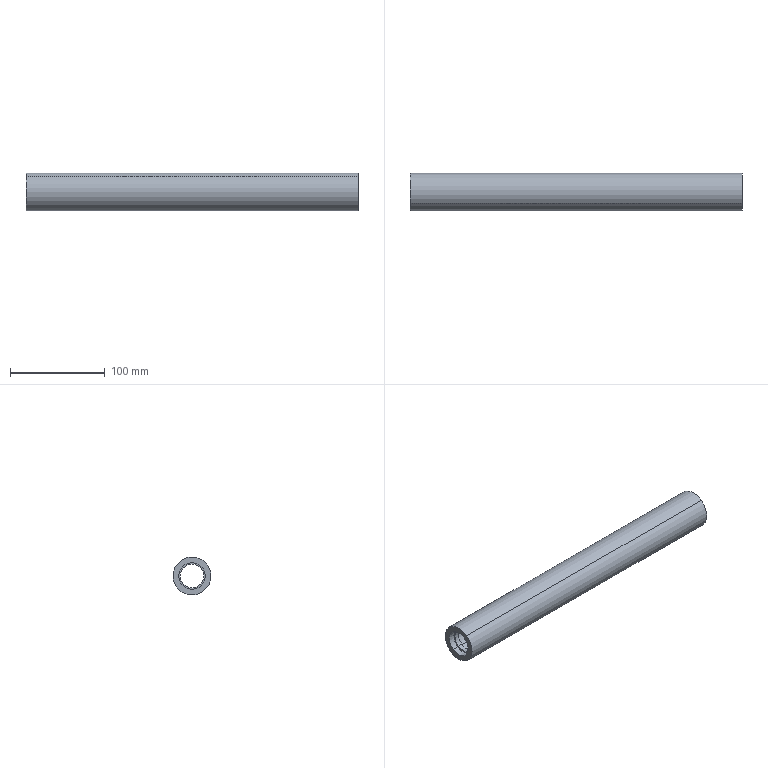Component | SolidWorks | 01-10MarkingMachineIdlerRoller-2 | 1 solid | 18 faces | box 350 x 40 x 40 mm | volume 130312 mm3 | cylinder 12 | plane 6 | commonest cylinder face diameters 28 x4 25 x4 40 x2 34 x2 | material A3 Steel
build123d program:
from build123d import *


with BuildPart() as part:
    # Sketch1 → Revolve1 (revolve)
    with BuildSketch(Plane.XY, mode=Mode.PRIVATE) as revolve1_sk:
        Polygon((-175, 20), (175, 20), (175, 14), (168, 14), (168, 12.5), (163, 12.5), (163, 17), (-163, 17), (-163, 12.5), (-168, 12.5), (-168, 14), (-175, 14), align=None)
    revolve(revolve1_sk.sketch.rotate(Axis((-220.554, 0, 0), (1, 0, 0)), 90), axis=Axis((-220.554, 0, 0), (1, 0, 0)))


solid = part.part

# Placed as in the assembly
solid = solid.moved(Location((-256.91, 57.41, 27.5), (0, 0, 0)))
STEP:
#1=COLOUR_RGB('',0.7922,0.8196,0.9333);
#2=FILL_AREA_STYLE_COLOUR('',#1);
#3=FILL_AREA_STYLE('',(#2));
#4=SURFACE_STYLE_FILL_AREA(#3);
#5=SURFACE_SIDE_STYLE('',(#4));
#6=SURFACE_STYLE_USAGE(.BOTH.,#5);
#7=PRESENTATION_STYLE_ASSIGNMENT((#6));
#8=CARTESIAN_POINT('',(-3.225,1.798,1.72));
#9=VERTEX_POINT('',#8);
#10=CARTESIAN_POINT('',(-3.225,2.722,0.4451));
#11=VERTEX_POINT('',#10);
#12=CARTESIAN_POINT('',(-3.225,2.26,1.083));
#13=DIRECTION('',(-1.,0.,0.));
#14=DIRECTION('',(0.,-0.5868,0.8097));
#15=AXIS2_PLACEMENT_3D('',#12,#13,#14);
#16=CIRCLE('',#15,0.7874);
#17=EDGE_CURVE('',#9,#11,#16,.T.);
#18=ORIENTED_EDGE('',*,*,#17,.T.);
#19=CARTESIAN_POINT('',(-17.004,2.722,0.4451));
#20=VERTEX_POINT('',#19);
#21=CARTESIAN_POINT('',(-18.798,2.722,0.4451));
#22=DIRECTION('',(-1.,0.,0.));
#23=VECTOR('',#22,39.37);
#24=LINE('',#21,#23);
#25=EDGE_CURVE('',#11,#20,#24,.T.);
#26=ORIENTED_EDGE('',*,*,#25,.T.);
#27=CARTESIAN_POINT('',(-17.004,1.798,1.72));
#28=VERTEX_POINT('',#27);
#29=CARTESIAN_POINT('',(-17.004,2.26,1.083));
#30=DIRECTION('',(-1.,0.,0.));
#31=DIRECTION('',(0.,-0.5868,0.8097));
#32=AXIS2_PLACEMENT_3D('',#29,#30,#31);
#33=CIRCLE('',#32,0.7874);
#34=EDGE_CURVE('',#28,#20,#33,.T.);
#35=ORIENTED_EDGE('',*,*,#34,.F.);
#36=CARTESIAN_POINT('',(-18.798,1.798,1.72));
#37=DIRECTION('',(-1.,0.,0.));
#38=VECTOR('',#37,39.37);
#39=LINE('',#36,#38);
#40=EDGE_CURVE('',#9,#28,#39,.T.);
#41=ORIENTED_EDGE('',*,*,#40,.F.);
#42=EDGE_LOOP('',(#18,#26,#35,#41));
#43=FACE_OUTER_BOUND('',#42,.T.);
#44=CARTESIAN_POINT('',(-18.798,2.26,1.083));
#45=DIRECTION('',(-1.,0.,0.));
#46=DIRECTION('',(0.,-0.5868,0.8097));
#47=AXIS2_PLACEMENT_3D('',#44,#45,#46);
#48=CYLINDRICAL_SURFACE('',#47,0.7874);
#49=ADVANCED_FACE('',(#43),#48,.T.);
#50=CARTESIAN_POINT('',(-3.225,2.584,0.6364));
#51=VERTEX_POINT('',#50);
#52=CARTESIAN_POINT('',(-3.225,1.937,1.529));
#53=VERTEX_POINT('',#52);
#54=CARTESIAN_POINT('',(-3.225,2.26,1.083));
#55=DIRECTION('',(-1.,0.,0.));
#56=DIRECTION('',(0.,-0.5868,0.8097));
#57=AXIS2_PLACEMENT_3D('',#54,#55,#56);
#58=CIRCLE('',#57,0.5512);
#59=EDGE_CURVE('',#51,#53,#58,.T.);
#60=ORIENTED_EDGE('',*,*,#59,.F.);
#61=CARTESIAN_POINT('',(-3.5,2.584,0.6364));
#62=VERTEX_POINT('',#61);
#63=CARTESIAN_POINT('',(-18.798,2.584,0.6364));
#64=DIRECTION('',(-1.,0.,0.));
#65=VECTOR('',#64,39.37);
#66=LINE('',#63,#65);
#67=EDGE_CURVE('',#51,#62,#66,.T.);
#68=ORIENTED_EDGE('',*,*,#67,.T.);
#69=CARTESIAN_POINT('',(-3.5,1.937,1.529));
#70=VERTEX_POINT('',#69);
#71=CARTESIAN_POINT('',(-3.5,2.26,1.083));
#72=DIRECTION('',(-1.,0.,0.));
#73=DIRECTION('',(0.,-0.5868,0.8097));
#74=AXIS2_PLACEMENT_3D('',#71,#72,#73);
#75=CIRCLE('',#74,0.5512);
#76=EDGE_CURVE('',#62,#70,#75,.T.);
#77=ORIENTED_EDGE('',*,*,#76,.T.);
#78=CARTESIAN_POINT('',(-18.798,1.937,1.529));
#79=DIRECTION('',(-1.,0.,0.));
#80=VECTOR('',#79,39.37);
#81=LINE('',#78,#80);
#82=EDGE_CURVE('',#53,#70,#81,.T.);
#83=ORIENTED_EDGE('',*,*,#82,.F.);
#84=EDGE_LOOP('',(#60,#68,#77,#83));
#85=FACE_OUTER_BOUND('',#84,.T.);
#86=CARTESIAN_POINT('',(-18.798,2.26,1.083));
#87=DIRECTION('',(-1.,0.,0.));
#88=DIRECTION('',(0.,-0.5868,0.8097));
#89=AXIS2_PLACEMENT_3D('',#86,#87,#88);
#90=CYLINDRICAL_SURFACE('',#89,0.5512);
#91=ADVANCED_FACE('',(#85),#90,.F.);
#92=CARTESIAN_POINT('',(-3.5,2.549,0.6842));
#93=VERTEX_POINT('',#92);
#94=CARTESIAN_POINT('',(-3.5,1.971,1.481));
#95=VERTEX_POINT('',#94);
#96=CARTESIAN_POINT('',(-3.5,2.26,1.083));
#97=DIRECTION('',(-1.,0.,0.));
#98=DIRECTION('',(0.,-0.5868,0.8097));
#99=AXIS2_PLACEMENT_3D('',#96,#97,#98);
#100=CIRCLE('',#99,0.4921);
#101=EDGE_CURVE('',#93,#95,#100,.T.);
#102=ORIENTED_EDGE('',*,*,#101,.F.);
#103=CARTESIAN_POINT('',(-3.697,2.549,0.6842));
#104=VERTEX_POINT('',#103);
#105=CARTESIAN_POINT('',(-18.798,2.549,0.6842));
#106=DIRECTION('',(-1.,0.,0.));
#107=VECTOR('',#106,39.37);
#108=LINE('',#105,#107);
#109=EDGE_CURVE('',#93,#104,#108,.T.);
#110=ORIENTED_EDGE('',*,*,#109,.T.);
#111=CARTESIAN_POINT('',(-3.697,1.971,1.481));
#112=VERTEX_POINT('',#111);
#113=CARTESIAN_POINT('',(-3.697,2.26,1.083));
#114=DIRECTION('',(-1.,0.,0.));
#115=DIRECTION('',(0.,-0.5868,0.8097));
#116=AXIS2_PLACEMENT_3D('',#113,#114,#115);
#117=CIRCLE('',#116,0.4921);
#118=EDGE_CURVE('',#104,#112,#117,.T.);
#119=ORIENTED_EDGE('',*,*,#118,.T.);
#120=CARTESIAN_POINT('',(-18.798,1.971,1.481));
#121=DIRECTION('',(-1.,0.,0.));
#122=VECTOR('',#121,39.37);
#123=LINE('',#120,#122);
#124=EDGE_CURVE('',#95,#112,#123,.T.);
#125=ORIENTED_EDGE('',*,*,#124,.F.);
#126=EDGE_LOOP('',(#102,#110,#119,#125));
#127=FACE_OUTER_BOUND('',#126,.T.);
#128=CARTESIAN_POINT('',(-18.798,2.26,1.083));
#129=DIRECTION('',(-1.,0.,0.));
#130=DIRECTION('',(0.,-0.5868,0.8097));
#131=AXIS2_PLACEMENT_3D('',#128,#129,#130);
#132=CYLINDRICAL_SURFACE('',#131,0.4921);
#133=ADVANCED_FACE('',(#127),#132,.F.);
#134=CARTESIAN_POINT('',(-3.697,2.653,0.5407));
#135=VERTEX_POINT('',#134);
#136=CARTESIAN_POINT('',(-3.697,1.867,1.625));
#137=VERTEX_POINT('',#136);
#138=CARTESIAN_POINT('',(-3.697,2.26,1.083));
#139=DIRECTION('',(-1.,0.,0.));
#140=DIRECTION('',(0.,-0.5868,0.8097));
#141=AXIS2_PLACEMENT_3D('',#138,#139,#140);
#142=CIRCLE('',#141,0.6693);
#143=EDGE_CURVE('',#135,#137,#142,.T.);
#144=ORIENTED_EDGE('',*,*,#143,.F.);
#145=CARTESIAN_POINT('',(-16.532,2.653,0.5407));
#146=VERTEX_POINT('',#145);
#147=CARTESIAN_POINT('',(-18.798,2.653,0.5407));
#148=DIRECTION('',(-1.,0.,0.));
#149=VECTOR('',#148,39.37);
#150=LINE('',#147,#149);
#151=EDGE_CURVE('',#135,#146,#150,.T.);
#152=ORIENTED_EDGE('',*,*,#151,.T.);
#153=CARTESIAN_POINT('',(-16.532,1.867,1.625));
#154=VERTEX_POINT('',#153);
#155=CARTESIAN_POINT('',(-16.532,2.26,1.083));
#156=DIRECTION('',(-1.,0.,0.));
#157=DIRECTION('',(0.,-0.5868,0.8097));
#158=AXIS2_PLACEMENT_3D('',#155,#156,#157);
#159=CIRCLE('',#158,0.6693);
#160=EDGE_CURVE('',#146,#154,#159,.T.);
#161=ORIENTED_EDGE('',*,*,#160,.T.);
#162=CARTESIAN_POINT('',(-18.798,1.867,1.625));
#163=DIRECTION('',(-1.,0.,0.));
#164=VECTOR('',#163,39.37);
#165=LINE('',#162,#164);
#166=EDGE_CURVE('',#137,#154,#165,.T.);
#167=ORIENTED_EDGE('',*,*,#166,.F.);
#168=EDGE_LOOP('',(#144,#152,#161,#167));
#169=FACE_OUTER_BOUND('',#168,.T.);
#170=CARTESIAN_POINT('',(-18.798,2.26,1.083));
#171=DIRECTION('',(-1.,0.,0.));
#172=DIRECTION('',(0.,-0.5868,0.8097));
#173=AXIS2_PLACEMENT_3D('',#170,#171,#172);
#174=CYLINDRICAL_SURFACE('',#173,0.6693);
#175=ADVANCED_FACE('',(#169),#174,.F.);
#176=CARTESIAN_POINT('',(-16.532,2.549,0.6842));
#177=VERTEX_POINT('',#176);
#178=CARTESIAN_POINT('',(-16.532,1.971,1.481));
#179=VERTEX_POINT('',#178);
#180=CARTESIAN_POINT('',(-16.532,2.26,1.083));
#181=DIRECTION('',(-1.,0.,0.));
#182=DIRECTION('',(0.,-0.5868,0.8097));
#183=AXIS2_PLACEMENT_3D('',#180,#181,#182);
#184=CIRCLE('',#183,0.4921);
#185=EDGE_CURVE('',#177,#179,#184,.T.);
#186=ORIENTED_EDGE('',*,*,#185,.F.);
#187=CARTESIAN_POINT('',(-16.729,2.549,0.6842));
#188=VERTEX_POINT('',#187);
#189=CARTESIAN_POINT('',(-18.798,2.549,0.6842));
#190=DIRECTION('',(-1.,0.,0.));
#191=VECTOR('',#190,39.37);
#192=LINE('',#189,#191);
#193=EDGE_CURVE('',#177,#188,#192,.T.);
#194=ORIENTED_EDGE('',*,*,#193,.T.);
#195=CARTESIAN_POINT('',(-16.729,1.971,1.481));
#196=VERTEX_POINT('',#195);
#197=CARTESIAN_POINT('',(-16.729,2.26,1.083));
#198=DIRECTION('',(-1.,0.,0.));
#199=DIRECTION('',(0.,-0.5868,0.8097));
#200=AXIS2_PLACEMENT_3D('',#197,#198,#199);
#201=CIRCLE('',#200,0.4921);
#202=EDGE_CURVE('',#188,#196,#201,.T.);
#203=ORIENTED_EDGE('',*,*,#202,.T.);
#204=CARTESIAN_POINT('',(-18.798,1.971,1.481));
#205=DIRECTION('',(-1.,0.,0.));
#206=VECTOR('',#205,39.37);
#207=LINE('',#204,#206);
#208=EDGE_CURVE('',#179,#196,#207,.T.);
#209=ORIENTED_EDGE('',*,*,#208,.F.);
#210=EDGE_LOOP('',(#186,#194,#203,#209));
#211=FACE_OUTER_BOUND('',#210,.T.);
#212=CARTESIAN_POINT('',(-18.798,2.26,1.083));
#213=DIRECTION('',(-1.,0.,0.));
#214=DIRECTION('',(0.,-0.5868,0.8097));
#215=AXIS2_PLACEMENT_3D('',#212,#213,#214);
#216=CYLINDRICAL_SURFACE('',#215,0.4921);
#217=ADVANCED_FACE('',(#211),#216,.F.);
#218=CARTESIAN_POINT('',(-16.729,2.584,0.6364));
#219=VERTEX_POINT('',#218);
#220=CARTESIAN_POINT('',(-16.729,1.937,1.529));
#221=VERTEX_POINT('',#220);
#222=CARTESIAN_POINT('',(-16.729,2.26,1.083));
#223=DIRECTION('',(-1.,0.,0.));
#224=DIRECTION('',(0.,-0.5868,0.8097));
#225=AXIS2_PLACEMENT_3D('',#222,#223,#224);
#226=CIRCLE('',#225,0.5512);
#227=EDGE_CURVE('',#219,#221,#226,.T.);
#228=ORIENTED_EDGE('',*,*,#227,.F.);
#229=CARTESIAN_POINT('',(-17.004,2.584,0.6364));
#230=VERTEX_POINT('',#229);
#231=CARTESIAN_POINT('',(-18.798,2.584,0.6364));
#232=DIRECTION('',(-1.,0.,0.));
#233=VECTOR('',#232,39.37);
#234=LINE('',#231,#233);
#235=EDGE_CURVE('',#219,#230,#234,.T.);
#236=ORIENTED_EDGE('',*,*,#235,.T.);
#237=CARTESIAN_POINT('',(-17.004,1.937,1.529));
#238=VERTEX_POINT('',#237);
#239=CARTESIAN_POINT('',(-17.004,2.26,1.083));
#240=DIRECTION('',(-1.,0.,0.));
#241=DIRECTION('',(0.,-0.5868,0.8097));
#242=AXIS2_PLACEMENT_3D('',#239,#240,#241);
#243=CIRCLE('',#242,0.5512);
#244=EDGE_CURVE('',#230,#238,#243,.T.);
#245=ORIENTED_EDGE('',*,*,#244,.T.);
#246=CARTESIAN_POINT('',(-18.798,1.937,1.529));
#247=DIRECTION('',(-1.,0.,0.));
#248=VECTOR('',#247,39.37);
#249=LINE('',#246,#248);
#250=EDGE_CURVE('',#221,#238,#249,.T.);
#251=ORIENTED_EDGE('',*,*,#250,.F.);
#252=EDGE_LOOP('',(#228,#236,#245,#251));
#253=FACE_OUTER_BOUND('',#252,.T.);
#254=CARTESIAN_POINT('',(-18.798,2.26,1.083));
#255=DIRECTION('',(-1.,0.,0.));
#256=DIRECTION('',(0.,-0.5868,0.8097));
#257=AXIS2_PLACEMENT_3D('',#254,#255,#256);
#258=CYLINDRICAL_SURFACE('',#257,0.5512);
#259=ADVANCED_FACE('',(#253),#258,.F.);
#260=CARTESIAN_POINT('',(-17.004,2.26,1.083));
#261=DIRECTION('',(-1.,0.,0.));
#262=DIRECTION('',(0.,-0.5868,0.8097));
#263=AXIS2_PLACEMENT_3D('',#260,#261,#262);
#264=CIRCLE('',#263,0.5512);
#265=EDGE_CURVE('',#238,#230,#264,.T.);
#266=ORIENTED_EDGE('',*,*,#265,.F.);
#267=ORIENTED_EDGE('',*,*,#244,.F.);
#268=EDGE_LOOP('',(#266,#267));
#269=FACE_BOUND('',#268,.T.);
#270=ORIENTED_EDGE('',*,*,#34,.T.);
#271=CARTESIAN_POINT('',(-17.004,2.26,1.083));
#272=DIRECTION('',(-1.,0.,0.));
#273=DIRECTION('',(0.,-0.5868,0.8097));
#274=AXIS2_PLACEMENT_3D('',#271,#272,#273);
#275=CIRCLE('',#274,0.7874);
#276=EDGE_CURVE('',#20,#28,#275,.T.);
#277=ORIENTED_EDGE('',*,*,#276,.T.);
#278=EDGE_LOOP('',(#270,#277));
#279=FACE_OUTER_BOUND('',#278,.T.);
#280=CARTESIAN_POINT('',(-17.004,2.898,1.545));
#281=DIRECTION('',(1.,0.,0.));
#282=DIRECTION('',(0.,0.5868,-0.8097));
#283=AXIS2_PLACEMENT_3D('',#280,#281,#282);
#284=PLANE('',#283);
#285=ADVANCED_FACE('',(#269,#279),#284,.F.);
#286=ORIENTED_EDGE('',*,*,#235,.F.);
#287=CARTESIAN_POINT('',(-16.729,2.26,1.083));
#288=DIRECTION('',(-1.,0.,0.));
#289=DIRECTION('',(0.,-0.5868,0.8097));
#290=AXIS2_PLACEMENT_3D('',#287,#288,#289);
#291=CIRCLE('',#290,0.5512);
#292=EDGE_CURVE('',#221,#219,#291,.T.);
#293=ORIENTED_EDGE('',*,*,#292,.F.);
#294=ORIENTED_EDGE('',*,*,#250,.T.);
#295=ORIENTED_EDGE('',*,*,#265,.T.);
#296=EDGE_LOOP('',(#286,#293,#294,#295));
#297=FACE_OUTER_BOUND('',#296,.T.);
#298=CARTESIAN_POINT('',(-18.798,2.26,1.083));
#299=DIRECTION('',(-1.,0.,0.));
#300=DIRECTION('',(0.,-0.5868,0.8097));
#301=AXIS2_PLACEMENT_3D('',#298,#299,#300);
#302=CYLINDRICAL_SURFACE('',#301,0.5512);
#303=ADVANCED_FACE('',(#297),#302,.F.);
#304=CARTESIAN_POINT('',(-16.729,2.26,1.083));
#305=DIRECTION('',(-1.,0.,0.));
#306=DIRECTION('',(0.,-0.5868,0.8097));
#307=AXIS2_PLACEMENT_3D('',#304,#305,#306);
#308=CIRCLE('',#307,0.4921);
#309=EDGE_CURVE('',#196,#188,#308,.T.);
#310=ORIENTED_EDGE('',*,*,#309,.F.);
#311=ORIENTED_EDGE('',*,*,#202,.F.);
#312=EDGE_LOOP('',(#310,#311));
#313=FACE_BOUND('',#312,.T.);
#314=ORIENTED_EDGE('',*,*,#292,.T.);
#315=ORIENTED_EDGE('',*,*,#227,.T.);
#316=EDGE_LOOP('',(#314,#315));
#317=FACE_OUTER_BOUND('',#316,.T.);
#318=CARTESIAN_POINT('',(-16.729,2.707,1.406));
#319=DIRECTION('',(1.,0.,0.));
#320=DIRECTION('',(0.,0.5868,-0.8097));
#321=AXIS2_PLACEMENT_3D('',#318,#319,#320);
#322=PLANE('',#321);
#323=ADVANCED_FACE('',(#313,#317),#322,.F.);
#324=ORIENTED_EDGE('',*,*,#193,.F.);
#325=CARTESIAN_POINT('',(-16.532,2.26,1.083));
#326=DIRECTION('',(-1.,0.,0.));
#327=DIRECTION('',(0.,-0.5868,0.8097));
#328=AXIS2_PLACEMENT_3D('',#325,#326,#327);
#329=CIRCLE('',#328,0.4921);
#330=EDGE_CURVE('',#179,#177,#329,.T.);
#331=ORIENTED_EDGE('',*,*,#330,.F.);
#332=ORIENTED_EDGE('',*,*,#208,.T.);
#333=ORIENTED_EDGE('',*,*,#309,.T.);
#334=EDGE_LOOP('',(#324,#331,#332,#333));
#335=FACE_OUTER_BOUND('',#334,.T.);
#336=CARTESIAN_POINT('',(-18.798,2.26,1.083));
#337=DIRECTION('',(-1.,0.,0.));
#338=DIRECTION('',(0.,-0.5868,0.8097));
#339=AXIS2_PLACEMENT_3D('',#336,#337,#338);
#340=CYLINDRICAL_SURFACE('',#339,0.4921);
#341=ADVANCED_FACE('',(#335),#340,.F.);
#342=CARTESIAN_POINT('',(-16.532,2.26,1.083));
#343=DIRECTION('',(-1.,0.,0.));
#344=DIRECTION('',(0.,-0.5868,0.8097));
#345=AXIS2_PLACEMENT_3D('',#342,#343,#344);
#346=CIRCLE('',#345,0.6693);
#347=EDGE_CURVE('',#154,#146,#346,.T.);
#348=ORIENTED_EDGE('',*,*,#347,.F.);
#349=ORIENTED_EDGE('',*,*,#160,.F.);
#350=EDGE_LOOP('',(#348,#349));
#351=FACE_OUTER_BOUND('',#350,.T.);
#352=ORIENTED_EDGE('',*,*,#330,.T.);
#353=ORIENTED_EDGE('',*,*,#185,.T.);
#354=EDGE_LOOP('',(#352,#353));
#355=FACE_BOUND('',#354,.T.);
#356=CARTESIAN_POINT('',(-16.532,2.659,1.371));
#357=DIRECTION('',(-1.,0.,0.));
#358=DIRECTION('',(0.,-0.5868,0.8097));
#359=AXIS2_PLACEMENT_3D('',#356,#357,#358);
#360=PLANE('',#359);
#361=ADVANCED_FACE('',(#351,#355),#360,.F.);
#362=ORIENTED_EDGE('',*,*,#151,.F.);
#363=CARTESIAN_POINT('',(-3.697,2.26,1.083));
#364=DIRECTION('',(-1.,0.,0.));
#365=DIRECTION('',(0.,-0.5868,0.8097));
#366=AXIS2_PLACEMENT_3D('',#363,#364,#365);
#367=CIRCLE('',#366,0.6693);
#368=EDGE_CURVE('',#137,#135,#367,.T.);
#369=ORIENTED_EDGE('',*,*,#368,.F.);
#370=ORIENTED_EDGE('',*,*,#166,.T.);
#371=ORIENTED_EDGE('',*,*,#347,.T.);
#372=EDGE_LOOP('',(#362,#369,#370,#371));
#373=FACE_OUTER_BOUND('',#372,.T.);
#374=CARTESIAN_POINT('',(-18.798,2.26,1.083));
#375=DIRECTION('',(-1.,0.,0.));
#376=DIRECTION('',(0.,-0.5868,0.8097));
#377=AXIS2_PLACEMENT_3D('',#374,#375,#376);
#378=CYLINDRICAL_SURFACE('',#377,0.6693);
#379=ADVANCED_FACE('',(#373),#378,.F.);
#380=CARTESIAN_POINT('',(-3.697,2.26,1.083));
#381=DIRECTION('',(-1.,0.,0.));
#382=DIRECTION('',(0.,-0.5868,0.8097));
#383=AXIS2_PLACEMENT_3D('',#380,#381,#382);
#384=CIRCLE('',#383,0.4921);
#385=EDGE_CURVE('',#112,#104,#384,.T.);
#386=ORIENTED_EDGE('',*,*,#385,.F.);
#387=ORIENTED_EDGE('',*,*,#118,.F.);
#388=EDGE_LOOP('',(#386,#387));
#389=FACE_BOUND('',#388,.T.);
#390=ORIENTED_EDGE('',*,*,#368,.T.);
#391=ORIENTED_EDGE('',*,*,#143,.T.);
#392=EDGE_LOOP('',(#390,#391));
#393=FACE_OUTER_BOUND('',#392,.T.);
#394=CARTESIAN_POINT('',(-3.697,2.659,1.371));
#395=DIRECTION('',(1.,0.,0.));
#396=DIRECTION('',(0.,0.5868,-0.8097));
#397=AXIS2_PLACEMENT_3D('',#394,#395,#396);
#398=PLANE('',#397);
#399=ADVANCED_FACE('',(#389,#393),#398,.F.);
#400=ORIENTED_EDGE('',*,*,#109,.F.);
#401=CARTESIAN_POINT('',(-3.5,2.26,1.083));
#402=DIRECTION('',(-1.,0.,0.));
#403=DIRECTION('',(0.,-0.5868,0.8097));
#404=AXIS2_PLACEMENT_3D('',#401,#402,#403);
#405=CIRCLE('',#404,0.4921);
#406=EDGE_CURVE('',#95,#93,#405,.T.);
#407=ORIENTED_EDGE('',*,*,#406,.F.);
#408=ORIENTED_EDGE('',*,*,#124,.T.);
#409=ORIENTED_EDGE('',*,*,#385,.T.);
#410=EDGE_LOOP('',(#400,#407,#408,#409));
#411=FACE_OUTER_BOUND('',#410,.T.);
#412=CARTESIAN_POINT('',(-18.798,2.26,1.083));
#413=DIRECTION('',(-1.,0.,0.));
#414=DIRECTION('',(0.,-0.5868,0.8097));
#415=AXIS2_PLACEMENT_3D('',#412,#413,#414);
#416=CYLINDRICAL_SURFACE('',#415,0.4921);
#417=ADVANCED_FACE('',(#411),#416,.F.);
#418=CARTESIAN_POINT('',(-3.5,2.26,1.083));
#419=DIRECTION('',(-1.,0.,0.));
#420=DIRECTION('',(0.,-0.5868,0.8097));
#421=AXIS2_PLACEMENT_3D('',#418,#419,#420);
#422=CIRCLE('',#421,0.5512);
#423=EDGE_CURVE('',#70,#62,#422,.T.);
#424=ORIENTED_EDGE('',*,*,#423,.F.);
#425=ORIENTED_EDGE('',*,*,#76,.F.);
#426=EDGE_LOOP('',(#424,#425));
#427=FACE_OUTER_BOUND('',#426,.T.);
#428=ORIENTED_EDGE('',*,*,#406,.T.);
#429=ORIENTED_EDGE('',*,*,#101,.T.);
#430=EDGE_LOOP('',(#428,#429));
#431=FACE_BOUND('',#430,.T.);
#432=CARTESIAN_POINT('',(-3.5,2.707,1.406));
#433=DIRECTION('',(-1.,0.,0.));
#434=DIRECTION('',(0.,-0.5868,0.8097));
#435=AXIS2_PLACEMENT_3D('',#432,#433,#434);
#436=PLANE('',#435);
#437=ADVANCED_FACE('',(#427,#431),#436,.F.);
#438=ORIENTED_EDGE('',*,*,#67,.F.);
#439=CARTESIAN_POINT('',(-3.225,2.26,1.083));
#440=DIRECTION('',(-1.,0.,0.));
#441=DIRECTION('',(0.,-0.5868,0.8097));
#442=AXIS2_PLACEMENT_3D('',#439,#440,#441);
#443=CIRCLE('',#442,0.5512);
#444=EDGE_CURVE('',#53,#51,#443,.T.);
#445=ORIENTED_EDGE('',*,*,#444,.F.);
#446=ORIENTED_EDGE('',*,*,#82,.T.);
#447=ORIENTED_EDGE('',*,*,#423,.T.);
#448=EDGE_LOOP('',(#438,#445,#446,#447));
#449=FACE_OUTER_BOUND('',#448,.T.);
#450=CARTESIAN_POINT('',(-18.798,2.26,1.083));
#451=DIRECTION('',(-1.,0.,0.));
#452=DIRECTION('',(0.,-0.5868,0.8097));
#453=AXIS2_PLACEMENT_3D('',#450,#451,#452);
#454=CYLINDRICAL_SURFACE('',#453,0.5512);
#455=ADVANCED_FACE('',(#449),#454,.F.);
#456=ORIENTED_EDGE('',*,*,#17,.F.);
#457=CARTESIAN_POINT('',(-3.225,2.26,1.083));
#458=DIRECTION('',(-1.,0.,0.));
#459=DIRECTION('',(0.,-0.5868,0.8097));
#460=AXIS2_PLACEMENT_3D('',#457,#458,#459);
#461=CIRCLE('',#460,0.7874);
#462=EDGE_CURVE('',#11,#9,#461,.T.);
#463=ORIENTED_EDGE('',*,*,#462,.F.);
#464=EDGE_LOOP('',(#456,#463));
#465=FACE_OUTER_BOUND('',#464,.T.);
#466=ORIENTED_EDGE('',*,*,#444,.T.);
#467=ORIENTED_EDGE('',*,*,#59,.T.);
#468=EDGE_LOOP('',(#466,#467));
#469=FACE_BOUND('',#468,.T.);
#470=CARTESIAN_POINT('',(-3.225,2.898,1.545));
#471=DIRECTION('',(-1.,0.,0.));
#472=DIRECTION('',(0.,-0.5868,0.8097));
#473=AXIS2_PLACEMENT_3D('',#470,#471,#472);
#474=PLANE('',#473);
#475=ADVANCED_FACE('',(#465,#469),#474,.F.);
#476=ORIENTED_EDGE('',*,*,#25,.F.);
#477=ORIENTED_EDGE('',*,*,#462,.T.);
#478=ORIENTED_EDGE('',*,*,#40,.T.);
#479=ORIENTED_EDGE('',*,*,#276,.F.);
#480=EDGE_LOOP('',(#476,#477,#478,#479));
#481=FACE_OUTER_BOUND('',#480,.T.);
#482=CARTESIAN_POINT('',(-18.798,2.26,1.083));
#483=DIRECTION('',(-1.,0.,0.));
#484=DIRECTION('',(0.,-0.5868,0.8097));
#485=AXIS2_PLACEMENT_3D('',#482,#483,#484);
#486=CYLINDRICAL_SURFACE('',#485,0.7874);
#487=ADVANCED_FACE('',(#481),#486,.T.);
#488=CLOSED_SHELL('',(#49,#91,#133,#175,#217,#259,#285,#303,#323,#341,#361,#379,#399,#417,#437,#455,#475,#487));
#489=MANIFOLD_SOLID_BREP('',#488);
#490=STYLED_ITEM('',(#7),#489);
#491=(LENGTH_UNIT()NAMED_UNIT(*)SI_UNIT($,.METRE.));
#492=LENGTH_MEASURE_WITH_UNIT(LENGTH_MEASURE(0.0254),#491);
#493=DIMENSIONAL_EXPONENTS(1.,0.,0.,0.,0.,0.,0.);
#494=(CONVERSION_BASED_UNIT('',#492)LENGTH_UNIT()NAMED_UNIT(#493));
#495=UNCERTAINTY_MEASURE_WITH_UNIT(LENGTH_MEASURE(0.00001),#494,'','');
#496=(NAMED_UNIT(*)PLANE_ANGLE_UNIT()SI_UNIT($,.RADIAN.));
#497=(NAMED_UNIT(*)SI_UNIT($,.STERADIAN.)SOLID_ANGLE_UNIT());
#498=(GEOMETRIC_REPRESENTATION_CONTEXT(3)GLOBAL_UNCERTAINTY_ASSIGNED_CONTEXT((#495))GLOBAL_UNIT_ASSIGNED_CONTEXT((#494,#496,#497))REPRESENTATION_CONTEXT('',''));
#499=MECHANICAL_DESIGN_GEOMETRIC_PRESENTATION_REPRESENTATION('',(#490),#498);
#500=CARTESIAN_POINT('',(0.,0.,0.));
#501=DIRECTION('',(0.,0.,1.));
#502=DIRECTION('',(1.,0.,0.));
#503=AXIS2_PLACEMENT_3D('',#500,#501,#502);
#504=(LENGTH_UNIT()NAMED_UNIT(*)SI_UNIT($,.METRE.));
#505=LENGTH_MEASURE_WITH_UNIT(LENGTH_MEASURE(0.0254),#504);
#506=DIMENSIONAL_EXPONENTS(1.,0.,0.,0.,0.,0.,0.);
#507=(CONVERSION_BASED_UNIT('',#505)LENGTH_UNIT()NAMED_UNIT(#506));
#508=UNCERTAINTY_MEASURE_WITH_UNIT(LENGTH_MEASURE(0.00001),#507,'','');
#509=(NAMED_UNIT(*)PLANE_ANGLE_UNIT()SI_UNIT($,.RADIAN.));
#510=(NAMED_UNIT(*)SI_UNIT($,.STERADIAN.)SOLID_ANGLE_UNIT());
#511=(GEOMETRIC_REPRESENTATION_CONTEXT(3)GLOBAL_UNCERTAINTY_ASSIGNED_CONTEXT((#508))GLOBAL_UNIT_ASSIGNED_CONTEXT((#507,#509,#510))REPRESENTATION_CONTEXT('',''));
#512=ADVANCED_BREP_SHAPE_REPRESENTATION('',(#489,#503),#511);
#513=PRESENTATION_LAYER_ASSIGNMENT('','',(#490));